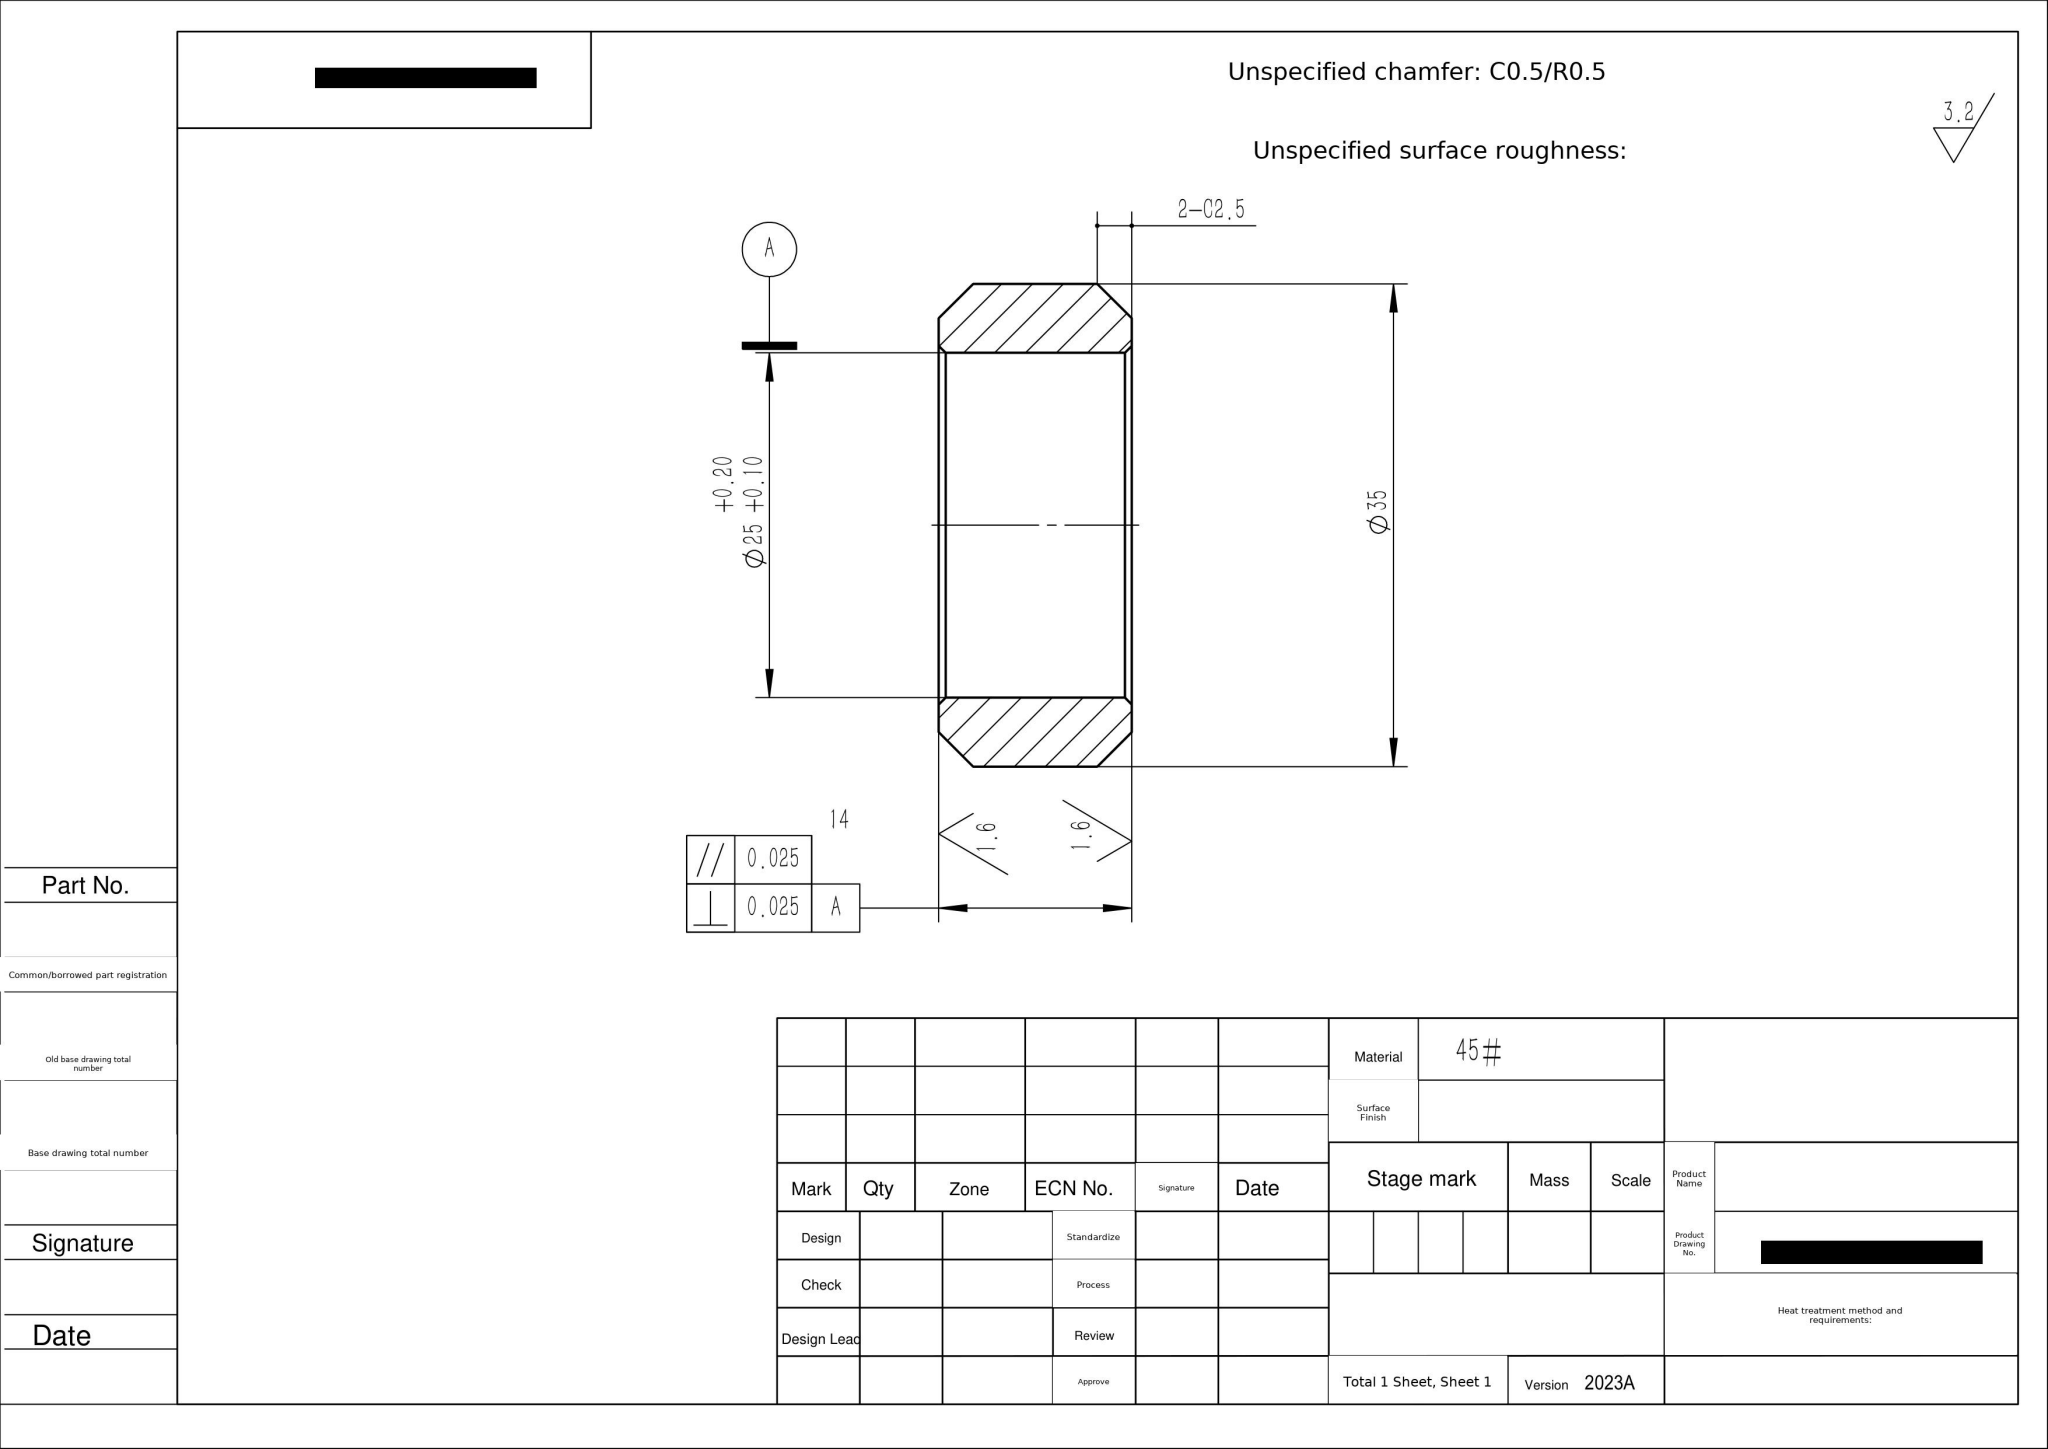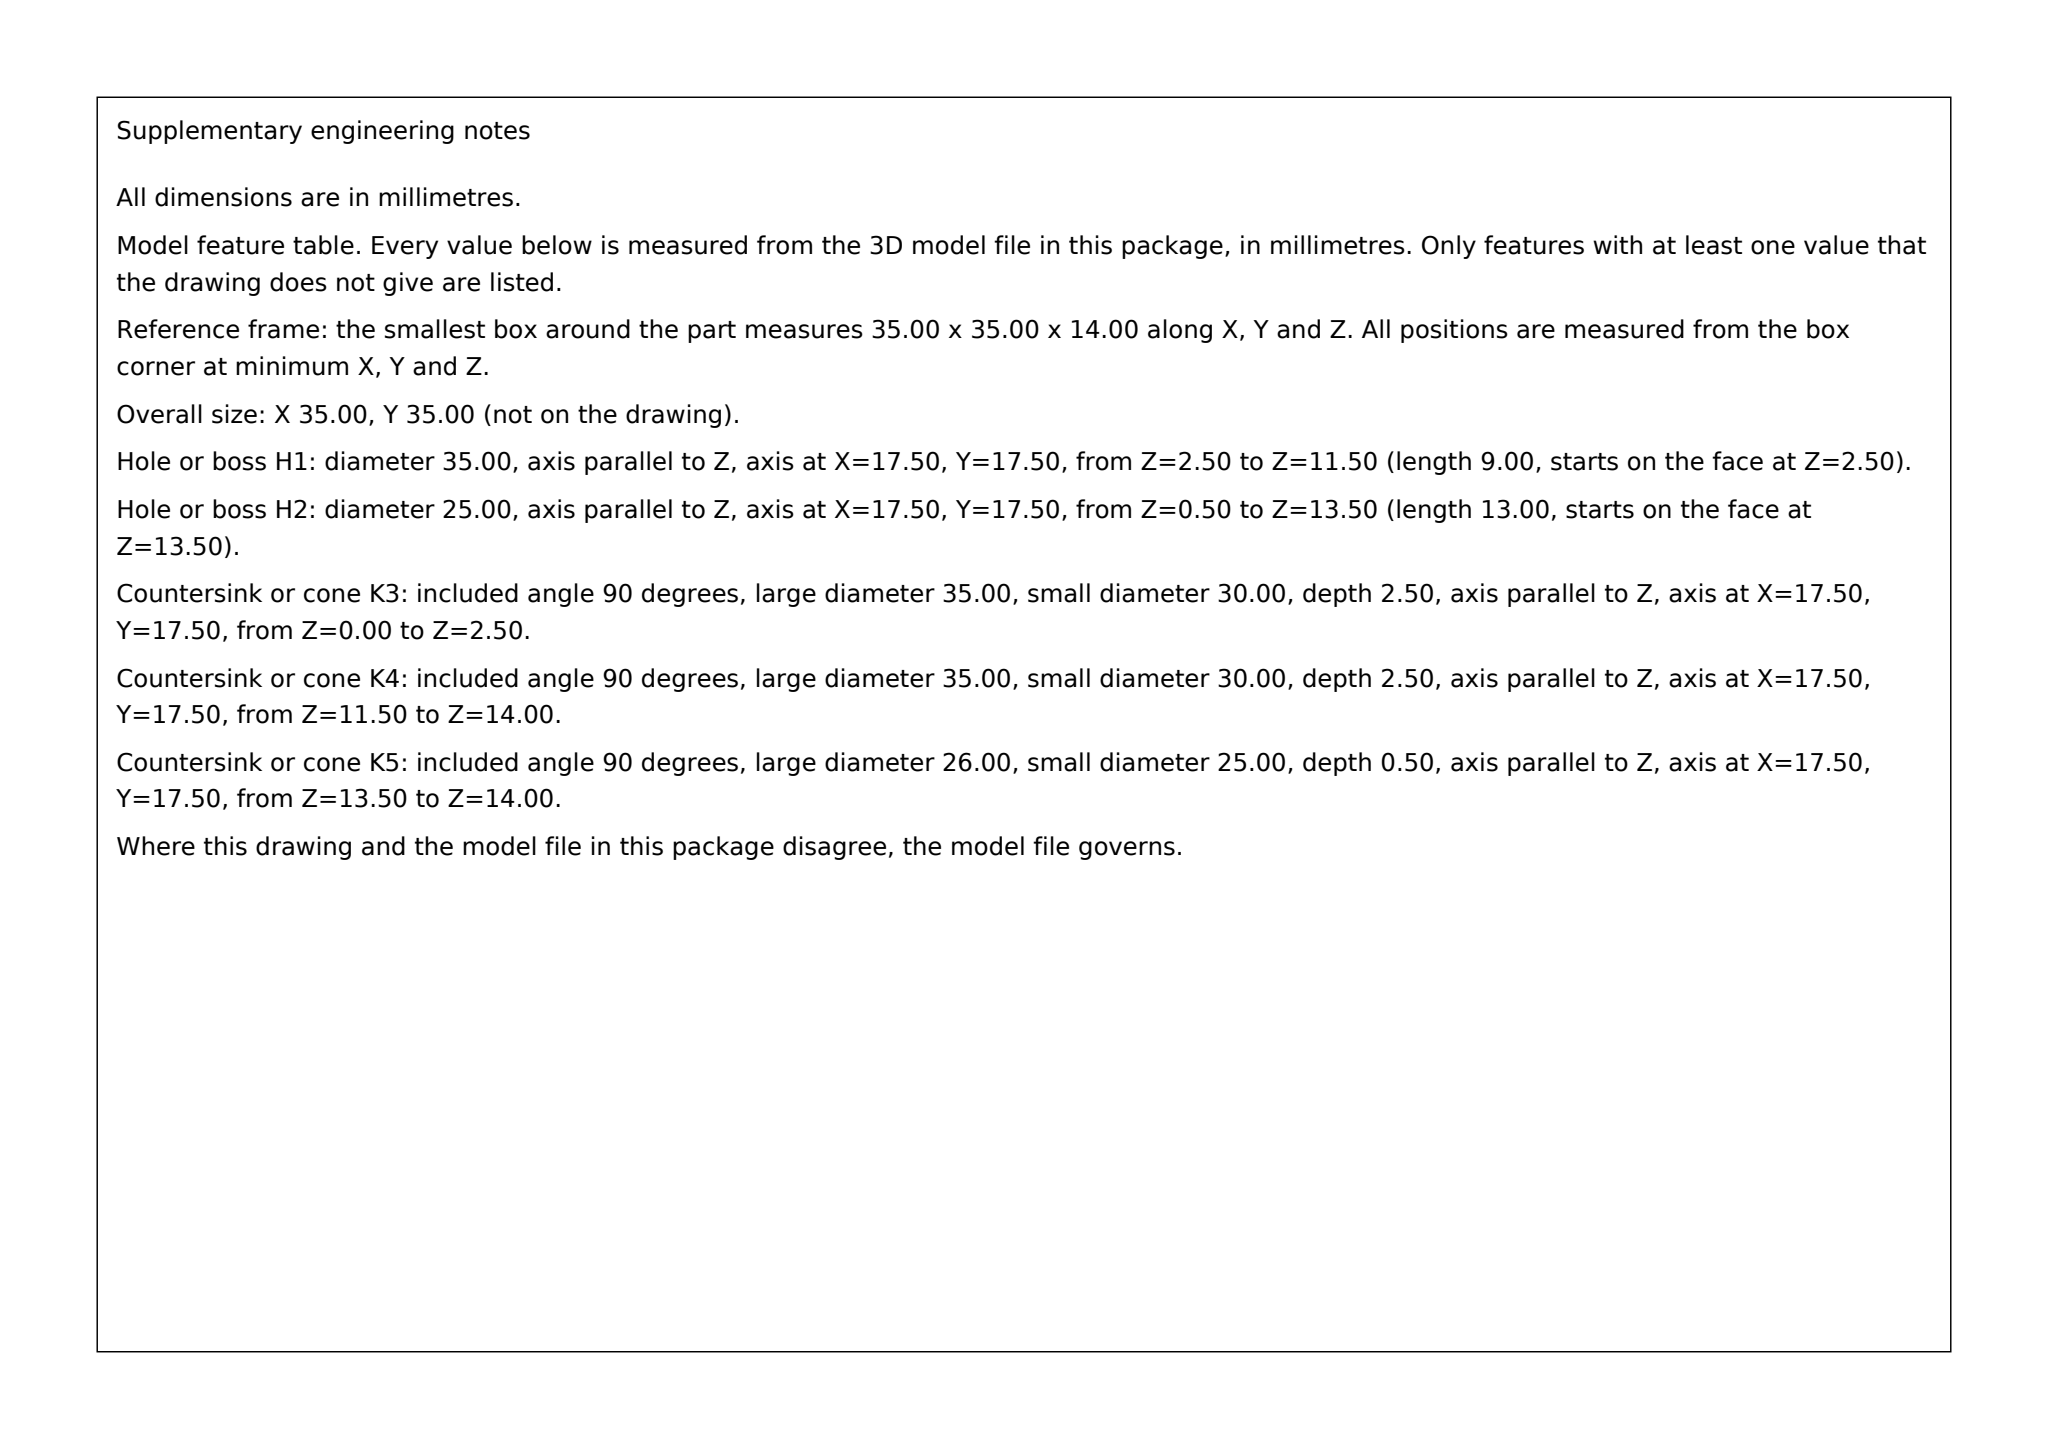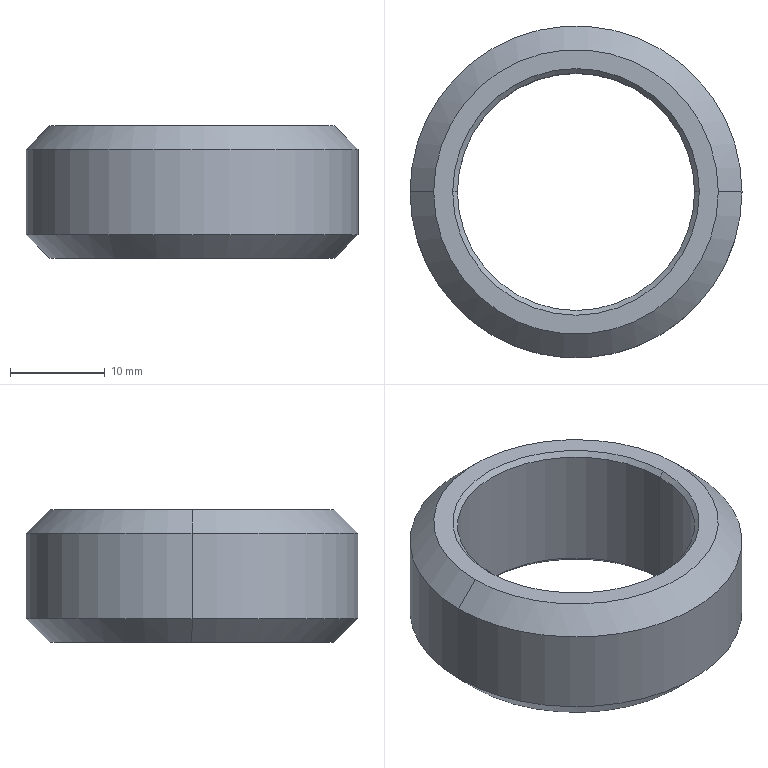Part | SolidWorks | mm | material 45# | 1 solid | 14 faces | box 35 x 35 x 14 mm | volume 5923 mm3 | cone 8 | cylinder 4 | plane 2 | commonest cylinder face diameters 25 x2 35 x2
build123d program:
from build123d import *

# Parameters (mm, degrees)
SKETCH1_R           = 17.5
SKETCH1_R_2         = 12.5
BOSS_EXTRUDE1_DEPTH = 14
CHAMFER1_SIZE       = 2.5
CHAMFER2_SIZE       = 0.5


with BuildPart() as part:
    # Sketch1 → Boss-Extrude1 (new body)
    with BuildSketch(Plane.XY):
        Circle(SKETCH1_R)
        Circle(SKETCH1_R_2, mode=Mode.SUBTRACT)
    extrude(amount=BOSS_EXTRUDE1_DEPTH)

    # Chamfer1
    chamfer1_edges = [part.edges().sort_by_distance(p)[0] for p in [
        (-17.5, 0, 0),
        (-17.5, 0, 14),
    ]]
    chamfer(chamfer1_edges, length=CHAMFER1_SIZE)

    # Chamfer2
    chamfer2_edges = [part.edges().sort_by_distance(p)[0] for p in [
        (-12.5, 0, 0),
        (-12.5, 0, 14),
    ]]
    chamfer(chamfer2_edges, length=CHAMFER2_SIZE)


solid = part.part
STEP:
#1=CARTESIAN_POINT('',(-12.5,0.,13.5));
#2=VERTEX_POINT('',#1);
#3=CARTESIAN_POINT('',(12.5,0.,13.5));
#4=VERTEX_POINT('',#3);
#5=CARTESIAN_POINT('',(0.,0.,13.5));
#6=DIRECTION('',(0.,0.,1.));
#7=DIRECTION('',(1.,0.,0.));
#8=AXIS2_PLACEMENT_3D('',#5,#6,#7);
#9=CIRCLE('',#8,12.5);
#10=EDGE_CURVE('',#2,#4,#9,.T.);
#11=ORIENTED_EDGE('',*,*,#10,.F.);
#12=CARTESIAN_POINT('',(-13.,0.,14.));
#13=VERTEX_POINT('',#12);
#14=CARTESIAN_POINT('',(-12.5,0.,13.5));
#15=DIRECTION('',(-0.7071,0.,0.7071));
#16=VECTOR('',#15,1000.);
#17=LINE('',#14,#16);
#18=EDGE_CURVE('',#2,#13,#17,.T.);
#19=ORIENTED_EDGE('',*,*,#18,.T.);
#20=CARTESIAN_POINT('',(13.,0.,14.));
#21=VERTEX_POINT('',#20);
#22=CARTESIAN_POINT('',(0.,0.,14.));
#23=DIRECTION('',(0.,0.,-1.));
#24=DIRECTION('',(1.,0.,0.));
#25=AXIS2_PLACEMENT_3D('',#22,#23,#24);
#26=CIRCLE('',#25,13.);
#27=EDGE_CURVE('',#21,#13,#26,.T.);
#28=ORIENTED_EDGE('',*,*,#27,.F.);
#29=CARTESIAN_POINT('',(12.5,0.,13.5));
#30=DIRECTION('',(0.7071,0.,0.7071));
#31=VECTOR('',#30,1000.);
#32=LINE('',#29,#31);
#33=EDGE_CURVE('',#4,#21,#32,.T.);
#34=ORIENTED_EDGE('',*,*,#33,.F.);
#35=EDGE_LOOP('',(#11,#19,#28,#34));
#36=FACE_OUTER_BOUND('',#35,.T.);
#37=CARTESIAN_POINT('',(0.,0.,13.5));
#38=DIRECTION('',(0.,0.,1.));
#39=DIRECTION('',(1.,0.,0.));
#40=AXIS2_PLACEMENT_3D('',#37,#38,#39);
#41=CONICAL_SURFACE('',#40,12.5,0.7854);
#42=ADVANCED_FACE('',(#36),#41,.F.);
#43=CARTESIAN_POINT('',(12.5,0.,0.5));
#44=VERTEX_POINT('',#43);
#45=CARTESIAN_POINT('',(-12.5,0.,0.5));
#46=VERTEX_POINT('',#45);
#47=CARTESIAN_POINT('',(0.,0.,0.5));
#48=DIRECTION('',(0.,0.,-1.));
#49=DIRECTION('',(1.,0.,0.));
#50=AXIS2_PLACEMENT_3D('',#47,#48,#49);
#51=CIRCLE('',#50,12.5);
#52=EDGE_CURVE('',#44,#46,#51,.T.);
#53=ORIENTED_EDGE('',*,*,#52,.F.);
#54=CARTESIAN_POINT('',(13.,0.,0.));
#55=VERTEX_POINT('',#54);
#56=CARTESIAN_POINT('',(13.,0.,0.));
#57=DIRECTION('',(0.7071,0.,-0.7071));
#58=VECTOR('',#57,1000.);
#59=LINE('',#56,#58);
#60=EDGE_CURVE('',#44,#55,#59,.T.);
#61=ORIENTED_EDGE('',*,*,#60,.T.);
#62=CARTESIAN_POINT('',(-13.,0.,0.));
#63=VERTEX_POINT('',#62);
#64=CARTESIAN_POINT('',(0.,0.,0.));
#65=DIRECTION('',(0.,0.,1.));
#66=DIRECTION('',(1.,0.,0.));
#67=AXIS2_PLACEMENT_3D('',#64,#65,#66);
#68=CIRCLE('',#67,13.);
#69=EDGE_CURVE('',#63,#55,#68,.T.);
#70=ORIENTED_EDGE('',*,*,#69,.F.);
#71=CARTESIAN_POINT('',(-13.,0.,0.));
#72=DIRECTION('',(-0.7071,0.,-0.7071));
#73=VECTOR('',#72,1000.);
#74=LINE('',#71,#73);
#75=EDGE_CURVE('',#46,#63,#74,.T.);
#76=ORIENTED_EDGE('',*,*,#75,.F.);
#77=EDGE_LOOP('',(#53,#61,#70,#76));
#78=FACE_OUTER_BOUND('',#77,.T.);
#79=CARTESIAN_POINT('',(0.,0.,0.));
#80=DIRECTION('',(0.,0.,-1.));
#81=DIRECTION('',(-1.,0.,0.));
#82=AXIS2_PLACEMENT_3D('',#79,#80,#81);
#83=CONICAL_SURFACE('',#82,13.,0.7854);
#84=ADVANCED_FACE('',(#78),#83,.F.);
#85=CARTESIAN_POINT('',(15.,0.,14.));
#86=VERTEX_POINT('',#85);
#87=CARTESIAN_POINT('',(-15.,0.,14.));
#88=VERTEX_POINT('',#87);
#89=CARTESIAN_POINT('',(0.,0.,14.));
#90=DIRECTION('',(0.,0.,1.));
#91=DIRECTION('',(1.,0.,0.));
#92=AXIS2_PLACEMENT_3D('',#89,#90,#91);
#93=CIRCLE('',#92,15.);
#94=EDGE_CURVE('',#86,#88,#93,.T.);
#95=ORIENTED_EDGE('',*,*,#94,.F.);
#96=CARTESIAN_POINT('',(17.5,0.,11.5));
#97=VERTEX_POINT('',#96);
#98=CARTESIAN_POINT('',(15.,0.,14.));
#99=DIRECTION('',(0.7071,0.,-0.7071));
#100=VECTOR('',#99,1000.);
#101=LINE('',#98,#100);
#102=EDGE_CURVE('',#86,#97,#101,.T.);
#103=ORIENTED_EDGE('',*,*,#102,.T.);
#104=CARTESIAN_POINT('',(-17.5,0.,11.5));
#105=VERTEX_POINT('',#104);
#106=CARTESIAN_POINT('',(0.,0.,11.5));
#107=DIRECTION('',(0.,0.,-1.));
#108=DIRECTION('',(1.,0.,0.));
#109=AXIS2_PLACEMENT_3D('',#106,#107,#108);
#110=CIRCLE('',#109,17.5);
#111=EDGE_CURVE('',#105,#97,#110,.T.);
#112=ORIENTED_EDGE('',*,*,#111,.F.);
#113=CARTESIAN_POINT('',(-15.,0.,14.));
#114=DIRECTION('',(-0.7071,0.,-0.7071));
#115=VECTOR('',#114,1000.);
#116=LINE('',#113,#115);
#117=EDGE_CURVE('',#88,#105,#116,.T.);
#118=ORIENTED_EDGE('',*,*,#117,.F.);
#119=EDGE_LOOP('',(#95,#103,#112,#118));
#120=FACE_OUTER_BOUND('',#119,.T.);
#121=CARTESIAN_POINT('',(0.,0.,14.));
#122=DIRECTION('',(0.,0.,-1.));
#123=DIRECTION('',(-1.,0.,0.));
#124=AXIS2_PLACEMENT_3D('',#121,#122,#123);
#125=CONICAL_SURFACE('',#124,15.,0.7854);
#126=ADVANCED_FACE('',(#120),#125,.T.);
#127=CARTESIAN_POINT('',(-15.,0.,0.));
#128=VERTEX_POINT('',#127);
#129=CARTESIAN_POINT('',(15.,0.,0.));
#130=VERTEX_POINT('',#129);
#131=CARTESIAN_POINT('',(0.,0.,0.));
#132=DIRECTION('',(0.,0.,-1.));
#133=DIRECTION('',(1.,0.,0.));
#134=AXIS2_PLACEMENT_3D('',#131,#132,#133);
#135=CIRCLE('',#134,15.);
#136=EDGE_CURVE('',#128,#130,#135,.T.);
#137=ORIENTED_EDGE('',*,*,#136,.F.);
#138=CARTESIAN_POINT('',(-17.5,0.,2.5));
#139=VERTEX_POINT('',#138);
#140=CARTESIAN_POINT('',(-17.5,0.,2.5));
#141=DIRECTION('',(-0.7071,0.,0.7071));
#142=VECTOR('',#141,1000.);
#143=LINE('',#140,#142);
#144=EDGE_CURVE('',#128,#139,#143,.T.);
#145=ORIENTED_EDGE('',*,*,#144,.T.);
#146=CARTESIAN_POINT('',(17.5,0.,2.5));
#147=VERTEX_POINT('',#146);
#148=CARTESIAN_POINT('',(0.,0.,2.5));
#149=DIRECTION('',(0.,0.,1.));
#150=DIRECTION('',(1.,0.,0.));
#151=AXIS2_PLACEMENT_3D('',#148,#149,#150);
#152=CIRCLE('',#151,17.5);
#153=EDGE_CURVE('',#147,#139,#152,.T.);
#154=ORIENTED_EDGE('',*,*,#153,.F.);
#155=CARTESIAN_POINT('',(17.5,0.,2.5));
#156=DIRECTION('',(0.7071,0.,0.7071));
#157=VECTOR('',#156,1000.);
#158=LINE('',#155,#157);
#159=EDGE_CURVE('',#130,#147,#158,.T.);
#160=ORIENTED_EDGE('',*,*,#159,.F.);
#161=EDGE_LOOP('',(#137,#145,#154,#160));
#162=FACE_OUTER_BOUND('',#161,.T.);
#163=CARTESIAN_POINT('',(0.,0.,2.5));
#164=DIRECTION('',(0.,0.,1.));
#165=DIRECTION('',(1.,0.,0.));
#166=AXIS2_PLACEMENT_3D('',#163,#164,#165);
#167=CONICAL_SURFACE('',#166,17.5,0.7854);
#168=ADVANCED_FACE('',(#162),#167,.T.);
#169=ORIENTED_EDGE('',*,*,#10,.T.);
#170=CARTESIAN_POINT('',(12.5,0.,14.));
#171=DIRECTION('',(0.,0.,-1.));
#172=VECTOR('',#171,1000.);
#173=LINE('',#170,#172);
#174=EDGE_CURVE('',#4,#44,#173,.T.);
#175=ORIENTED_EDGE('',*,*,#174,.T.);
#176=ORIENTED_EDGE('',*,*,#52,.T.);
#177=CARTESIAN_POINT('',(-12.5,0.,14.));
#178=DIRECTION('',(0.,0.,-1.));
#179=VECTOR('',#178,1000.);
#180=LINE('',#177,#179);
#181=EDGE_CURVE('',#2,#46,#180,.T.);
#182=ORIENTED_EDGE('',*,*,#181,.F.);
#183=EDGE_LOOP('',(#169,#175,#176,#182));
#184=FACE_OUTER_BOUND('',#183,.T.);
#185=CARTESIAN_POINT('',(0.,0.,14.));
#186=DIRECTION('',(0.,0.,-1.));
#187=DIRECTION('',(-1.,0.,0.));
#188=AXIS2_PLACEMENT_3D('',#185,#186,#187);
#189=CYLINDRICAL_SURFACE('',#188,12.5);
#190=ADVANCED_FACE('',(#184),#189,.F.);
#191=ORIENTED_EDGE('',*,*,#111,.T.);
#192=CARTESIAN_POINT('',(17.5,0.,14.));
#193=DIRECTION('',(0.,0.,-1.));
#194=VECTOR('',#193,1000.);
#195=LINE('',#192,#194);
#196=EDGE_CURVE('',#97,#147,#195,.T.);
#197=ORIENTED_EDGE('',*,*,#196,.T.);
#198=ORIENTED_EDGE('',*,*,#153,.T.);
#199=CARTESIAN_POINT('',(-17.5,0.,14.));
#200=DIRECTION('',(0.,0.,-1.));
#201=VECTOR('',#200,1000.);
#202=LINE('',#199,#201);
#203=EDGE_CURVE('',#105,#139,#202,.T.);
#204=ORIENTED_EDGE('',*,*,#203,.F.);
#205=EDGE_LOOP('',(#191,#197,#198,#204));
#206=FACE_OUTER_BOUND('',#205,.T.);
#207=CARTESIAN_POINT('',(0.,0.,14.));
#208=DIRECTION('',(0.,0.,-1.));
#209=DIRECTION('',(-1.,0.,0.));
#210=AXIS2_PLACEMENT_3D('',#207,#208,#209);
#211=CYLINDRICAL_SURFACE('',#210,17.5);
#212=ADVANCED_FACE('',(#206),#211,.T.);
#213=ORIENTED_EDGE('',*,*,#27,.T.);
#214=CARTESIAN_POINT('',(0.,0.,14.));
#215=DIRECTION('',(0.,0.,-1.));
#216=DIRECTION('',(1.,0.,0.));
#217=AXIS2_PLACEMENT_3D('',#214,#215,#216);
#218=CIRCLE('',#217,13.);
#219=EDGE_CURVE('',#13,#21,#218,.T.);
#220=ORIENTED_EDGE('',*,*,#219,.T.);
#221=EDGE_LOOP('',(#213,#220));
#222=FACE_BOUND('',#221,.T.);
#223=CARTESIAN_POINT('',(0.,0.,14.));
#224=DIRECTION('',(0.,0.,1.));
#225=DIRECTION('',(1.,0.,0.));
#226=AXIS2_PLACEMENT_3D('',#223,#224,#225);
#227=CIRCLE('',#226,15.);
#228=EDGE_CURVE('',#88,#86,#227,.T.);
#229=ORIENTED_EDGE('',*,*,#228,.T.);
#230=ORIENTED_EDGE('',*,*,#94,.T.);
#231=EDGE_LOOP('',(#229,#230));
#232=FACE_OUTER_BOUND('',#231,.T.);
#233=CARTESIAN_POINT('',(0.,0.,14.));
#234=DIRECTION('',(0.,0.,1.));
#235=DIRECTION('',(1.,0.,0.));
#236=AXIS2_PLACEMENT_3D('',#233,#234,#235);
#237=PLANE('',#236);
#238=ADVANCED_FACE('',(#222,#232),#237,.T.);
#239=ORIENTED_EDGE('',*,*,#69,.T.);
#240=CARTESIAN_POINT('',(0.,0.,0.));
#241=DIRECTION('',(0.,0.,1.));
#242=DIRECTION('',(1.,0.,0.));
#243=AXIS2_PLACEMENT_3D('',#240,#241,#242);
#244=CIRCLE('',#243,13.);
#245=EDGE_CURVE('',#55,#63,#244,.T.);
#246=ORIENTED_EDGE('',*,*,#245,.T.);
#247=EDGE_LOOP('',(#239,#246));
#248=FACE_BOUND('',#247,.T.);
#249=CARTESIAN_POINT('',(0.,0.,0.));
#250=DIRECTION('',(0.,0.,-1.));
#251=DIRECTION('',(1.,0.,0.));
#252=AXIS2_PLACEMENT_3D('',#249,#250,#251);
#253=CIRCLE('',#252,15.);
#254=EDGE_CURVE('',#130,#128,#253,.T.);
#255=ORIENTED_EDGE('',*,*,#254,.T.);
#256=ORIENTED_EDGE('',*,*,#136,.T.);
#257=EDGE_LOOP('',(#255,#256));
#258=FACE_OUTER_BOUND('',#257,.T.);
#259=CARTESIAN_POINT('',(0.,0.,0.));
#260=DIRECTION('',(0.,0.,1.));
#261=DIRECTION('',(1.,0.,0.));
#262=AXIS2_PLACEMENT_3D('',#259,#260,#261);
#263=PLANE('',#262);
#264=ADVANCED_FACE('',(#248,#258),#263,.F.);
#265=ORIENTED_EDGE('',*,*,#196,.F.);
#266=CARTESIAN_POINT('',(0.,0.,11.5));
#267=DIRECTION('',(0.,0.,-1.));
#268=DIRECTION('',(1.,0.,0.));
#269=AXIS2_PLACEMENT_3D('',#266,#267,#268);
#270=CIRCLE('',#269,17.5);
#271=EDGE_CURVE('',#97,#105,#270,.T.);
#272=ORIENTED_EDGE('',*,*,#271,.T.);
#273=ORIENTED_EDGE('',*,*,#203,.T.);
#274=CARTESIAN_POINT('',(0.,0.,2.5));
#275=DIRECTION('',(0.,0.,1.));
#276=DIRECTION('',(1.,0.,0.));
#277=AXIS2_PLACEMENT_3D('',#274,#275,#276);
#278=CIRCLE('',#277,17.5);
#279=EDGE_CURVE('',#139,#147,#278,.T.);
#280=ORIENTED_EDGE('',*,*,#279,.T.);
#281=EDGE_LOOP('',(#265,#272,#273,#280));
#282=FACE_OUTER_BOUND('',#281,.T.);
#283=CARTESIAN_POINT('',(0.,0.,14.));
#284=DIRECTION('',(0.,0.,-1.));
#285=DIRECTION('',(-1.,0.,0.));
#286=AXIS2_PLACEMENT_3D('',#283,#284,#285);
#287=CYLINDRICAL_SURFACE('',#286,17.5);
#288=ADVANCED_FACE('',(#282),#287,.T.);
#289=ORIENTED_EDGE('',*,*,#174,.F.);
#290=CARTESIAN_POINT('',(0.,0.,13.5));
#291=DIRECTION('',(0.,0.,1.));
#292=DIRECTION('',(1.,0.,0.));
#293=AXIS2_PLACEMENT_3D('',#290,#291,#292);
#294=CIRCLE('',#293,12.5);
#295=EDGE_CURVE('',#4,#2,#294,.T.);
#296=ORIENTED_EDGE('',*,*,#295,.T.);
#297=ORIENTED_EDGE('',*,*,#181,.T.);
#298=CARTESIAN_POINT('',(0.,0.,0.5));
#299=DIRECTION('',(0.,0.,-1.));
#300=DIRECTION('',(1.,0.,0.));
#301=AXIS2_PLACEMENT_3D('',#298,#299,#300);
#302=CIRCLE('',#301,12.5);
#303=EDGE_CURVE('',#46,#44,#302,.T.);
#304=ORIENTED_EDGE('',*,*,#303,.T.);
#305=EDGE_LOOP('',(#289,#296,#297,#304));
#306=FACE_OUTER_BOUND('',#305,.T.);
#307=CARTESIAN_POINT('',(0.,0.,14.));
#308=DIRECTION('',(0.,0.,-1.));
#309=DIRECTION('',(-1.,0.,0.));
#310=AXIS2_PLACEMENT_3D('',#307,#308,#309);
#311=CYLINDRICAL_SURFACE('',#310,12.5);
#312=ADVANCED_FACE('',(#306),#311,.F.);
#313=ORIENTED_EDGE('',*,*,#144,.F.);
#314=ORIENTED_EDGE('',*,*,#254,.F.);
#315=ORIENTED_EDGE('',*,*,#159,.T.);
#316=ORIENTED_EDGE('',*,*,#279,.F.);
#317=EDGE_LOOP('',(#313,#314,#315,#316));
#318=FACE_OUTER_BOUND('',#317,.T.);
#319=CARTESIAN_POINT('',(0.,0.,2.5));
#320=DIRECTION('',(0.,0.,1.));
#321=DIRECTION('',(1.,0.,0.));
#322=AXIS2_PLACEMENT_3D('',#319,#320,#321);
#323=CONICAL_SURFACE('',#322,17.5,0.7854);
#324=ADVANCED_FACE('',(#318),#323,.T.);
#325=ORIENTED_EDGE('',*,*,#102,.F.);
#326=ORIENTED_EDGE('',*,*,#228,.F.);
#327=ORIENTED_EDGE('',*,*,#117,.T.);
#328=ORIENTED_EDGE('',*,*,#271,.F.);
#329=EDGE_LOOP('',(#325,#326,#327,#328));
#330=FACE_OUTER_BOUND('',#329,.T.);
#331=CARTESIAN_POINT('',(0.,0.,14.));
#332=DIRECTION('',(0.,0.,-1.));
#333=DIRECTION('',(-1.,0.,0.));
#334=AXIS2_PLACEMENT_3D('',#331,#332,#333);
#335=CONICAL_SURFACE('',#334,15.,0.7854);
#336=ADVANCED_FACE('',(#330),#335,.T.);
#337=ORIENTED_EDGE('',*,*,#60,.F.);
#338=ORIENTED_EDGE('',*,*,#303,.F.);
#339=ORIENTED_EDGE('',*,*,#75,.T.);
#340=ORIENTED_EDGE('',*,*,#245,.F.);
#341=EDGE_LOOP('',(#337,#338,#339,#340));
#342=FACE_OUTER_BOUND('',#341,.T.);
#343=CARTESIAN_POINT('',(0.,0.,0.));
#344=DIRECTION('',(0.,0.,-1.));
#345=DIRECTION('',(-1.,0.,0.));
#346=AXIS2_PLACEMENT_3D('',#343,#344,#345);
#347=CONICAL_SURFACE('',#346,13.,0.7854);
#348=ADVANCED_FACE('',(#342),#347,.F.);
#349=ORIENTED_EDGE('',*,*,#18,.F.);
#350=ORIENTED_EDGE('',*,*,#295,.F.);
#351=ORIENTED_EDGE('',*,*,#33,.T.);
#352=ORIENTED_EDGE('',*,*,#219,.F.);
#353=EDGE_LOOP('',(#349,#350,#351,#352));
#354=FACE_OUTER_BOUND('',#353,.T.);
#355=CARTESIAN_POINT('',(0.,0.,13.5));
#356=DIRECTION('',(0.,0.,1.));
#357=DIRECTION('',(1.,0.,0.));
#358=AXIS2_PLACEMENT_3D('',#355,#356,#357);
#359=CONICAL_SURFACE('',#358,12.5,0.7854);
#360=ADVANCED_FACE('',(#354),#359,.F.);
#361=CLOSED_SHELL('',(#42,#84,#126,#168,#190,#212,#238,#264,#288,#312,#324,#336,#348,#360));
#362=MANIFOLD_SOLID_BREP('',#361);
#363=CARTESIAN_POINT('',(0.,0.,0.));
#364=DIRECTION('',(0.,0.,1.));
#365=DIRECTION('',(1.,0.,0.));
#366=AXIS2_PLACEMENT_3D('',#363,#364,#365);
#367=(LENGTH_UNIT()NAMED_UNIT(*)SI_UNIT(.MILLI.,.METRE.));
#368=UNCERTAINTY_MEASURE_WITH_UNIT(LENGTH_MEASURE(0.00001),#367,'','');
#369=(NAMED_UNIT(*)PLANE_ANGLE_UNIT()SI_UNIT($,.RADIAN.));
#370=(NAMED_UNIT(*)SI_UNIT($,.STERADIAN.)SOLID_ANGLE_UNIT());
#371=(GEOMETRIC_REPRESENTATION_CONTEXT(3)GLOBAL_UNCERTAINTY_ASSIGNED_CONTEXT((#368))GLOBAL_UNIT_ASSIGNED_CONTEXT((#367,#369,#370))REPRESENTATION_CONTEXT('',''));
#372=ADVANCED_BREP_SHAPE_REPRESENTATION('',(#362,#366),#371);